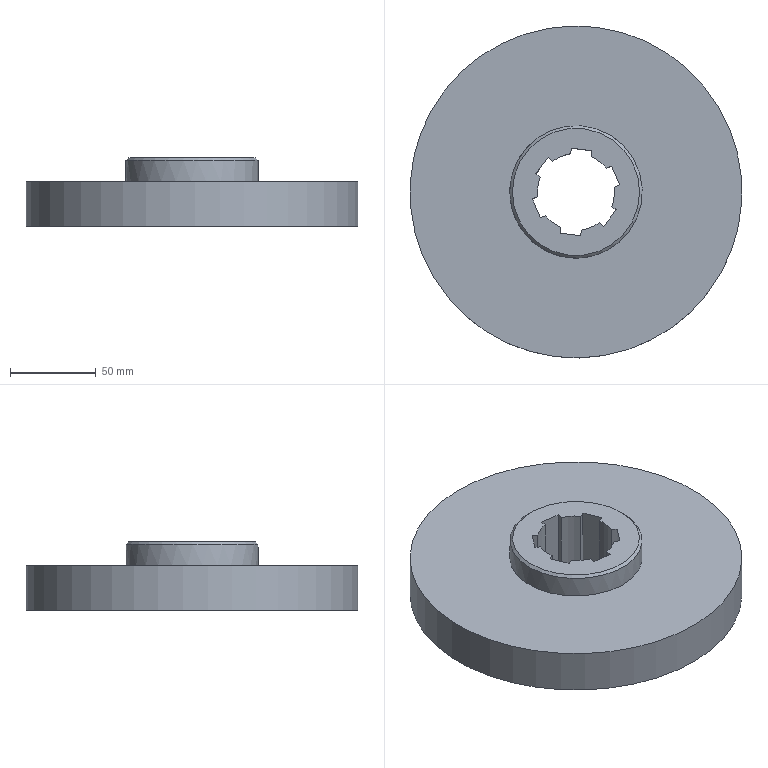Component | NX | ZHOUV2 | 1 solid | 30 faces | volume 760305 mm3 | plane 21 | cylinder 8 | cone 1 | commonest cylinder face diameters 45 x6 193.75 x1 77.253 x1